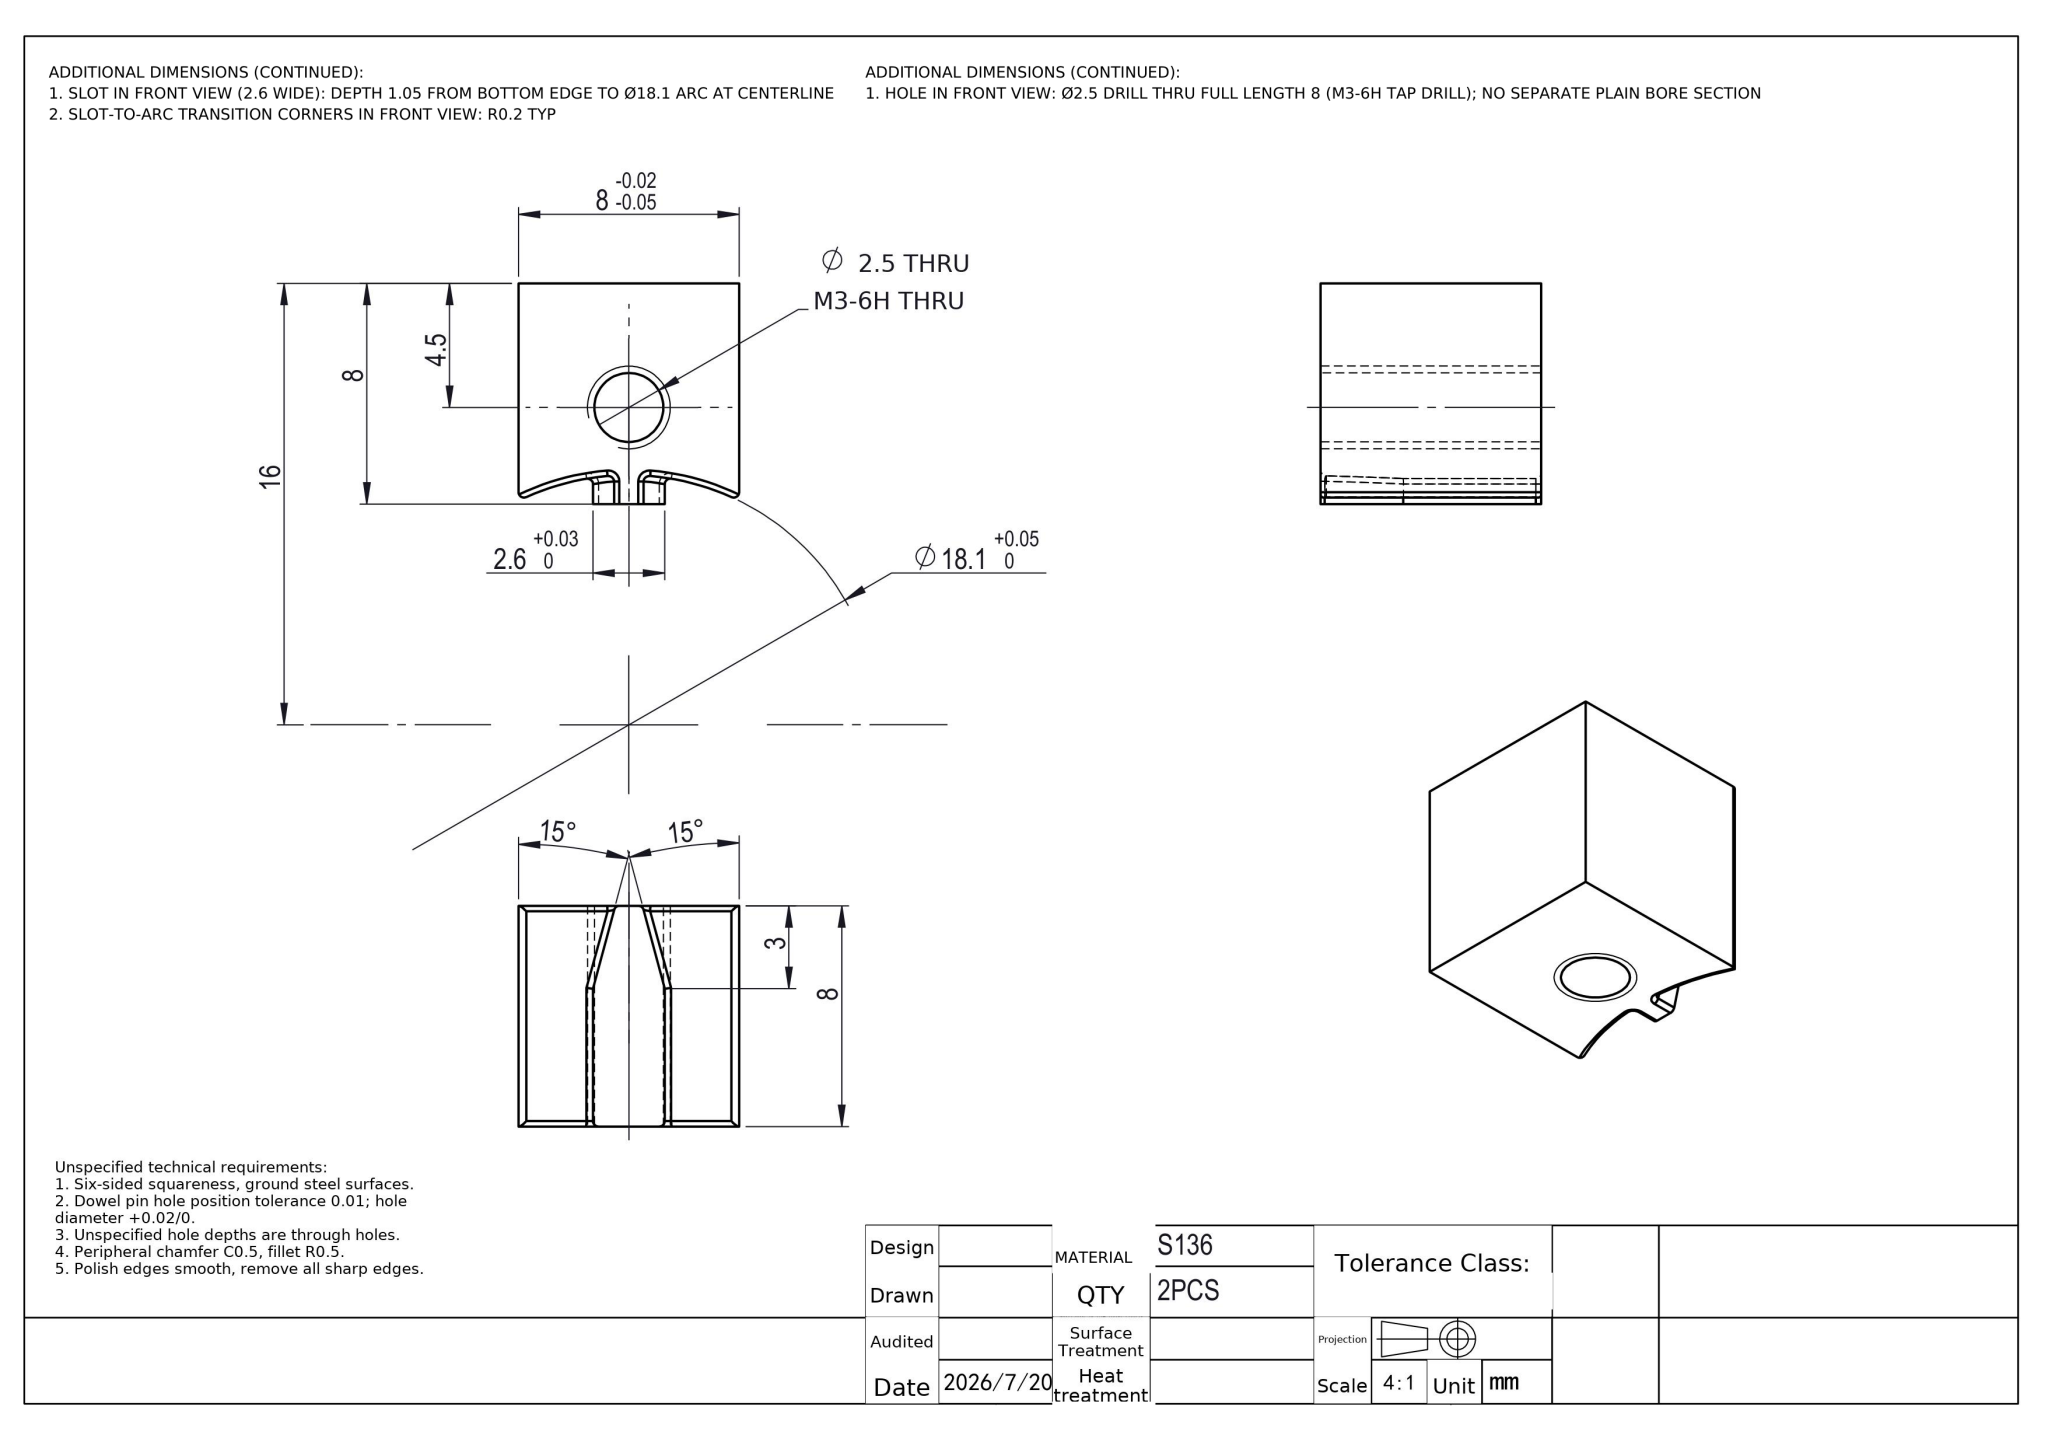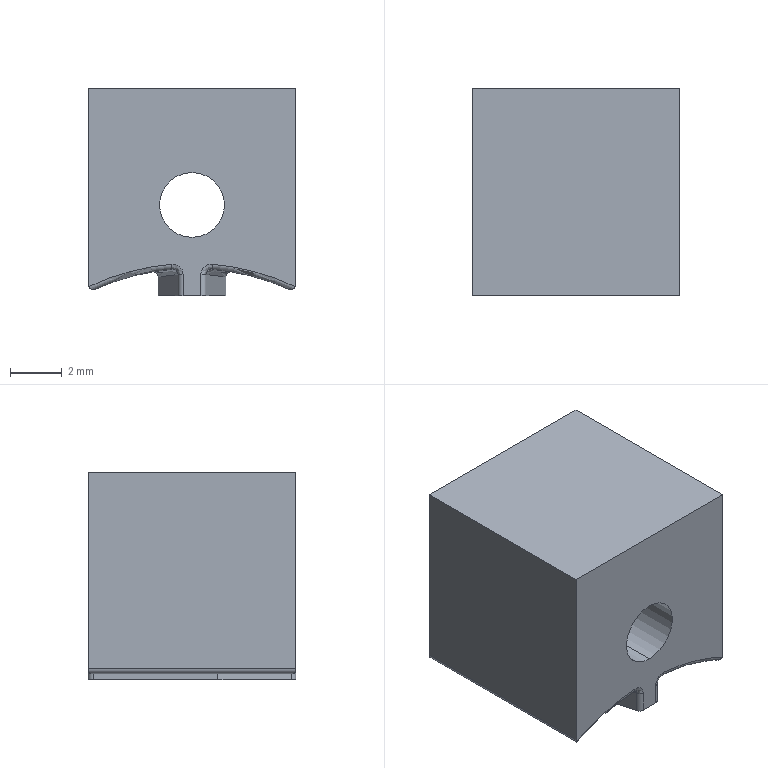Part | NX | mm | 1 solid | 34 faces | box 8 x 8 x 8 mm | volume 443 mm3 | cylinder 14 | plane 10 | torus 6 | spline 4 | commonest cylinder face diameters 0.4 x10 2.5 x2 18.1 x2